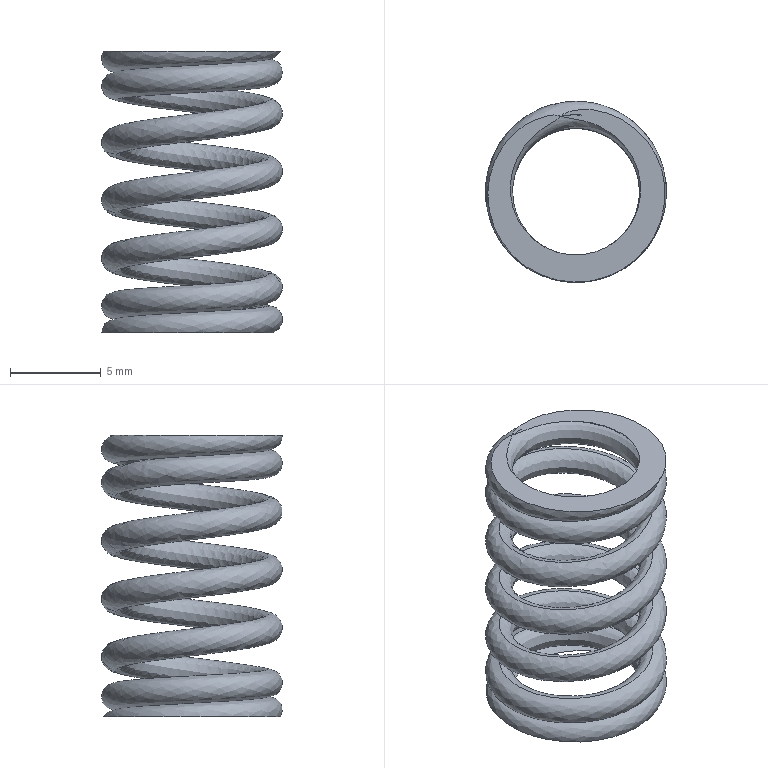Component | SolidWorks | OuterDiameter10WireDiameter1Height20CompressionSpring-1 | 1 solid | 4 faces | volume 297 mm3 | spline 2 | plane 2 | material A3 Steel